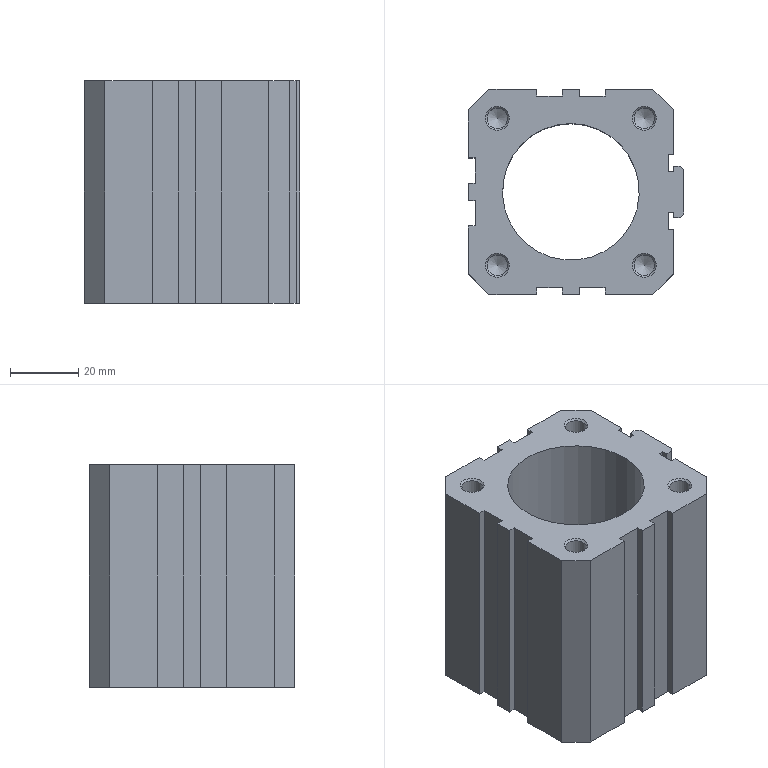Component | NX | CYLINDER | 1 solid | 73 faces | volume 141371 mm3 | plane 48 | cone 16 | cylinder 9 | commonest cylinder face diameters 5 x4 6 x4 40 x1